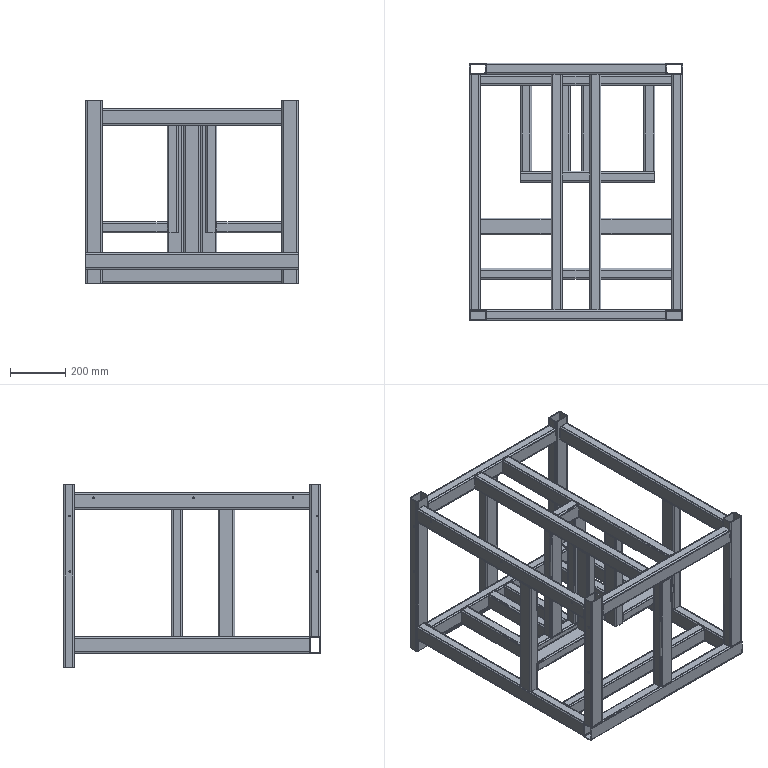Component | SolidWorks | STE21014.01-01-1 | 32 solids | 608 faces | volume 10043338 mm3 | plane 320 | cylinder 288 | commonest cylinder face diameters 6.4 x128 12.8 x128 6.8 x32 | material Q235